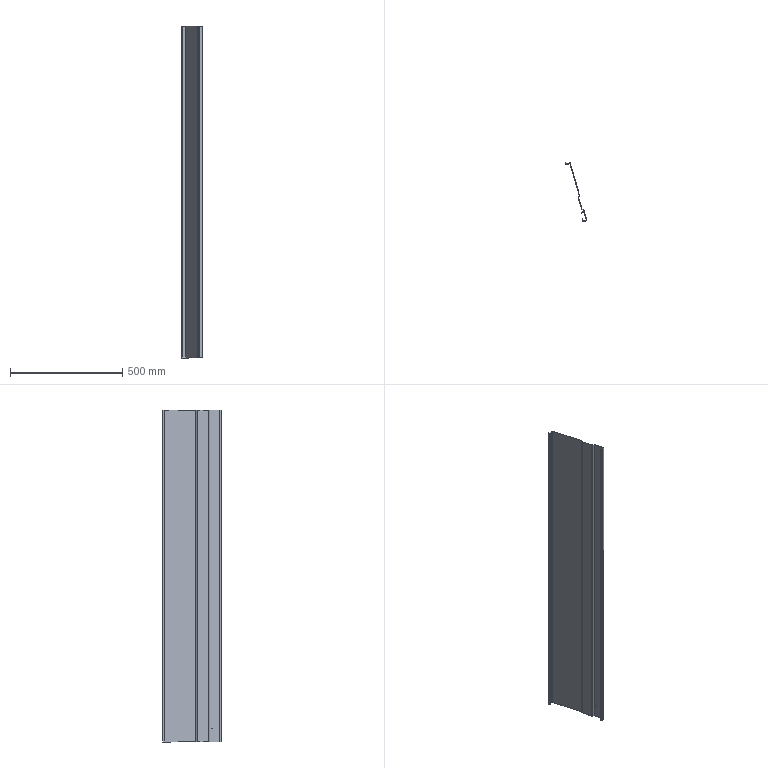Component | SolidWorks | LeftDoorAssembly-1_LeftDoor-1 | 1 solid | 73 faces | volume 708851 mm3 | plane 55 | cylinder 18 | commonest cylinder face diameters 2 x8 5 x8 4.1 x2